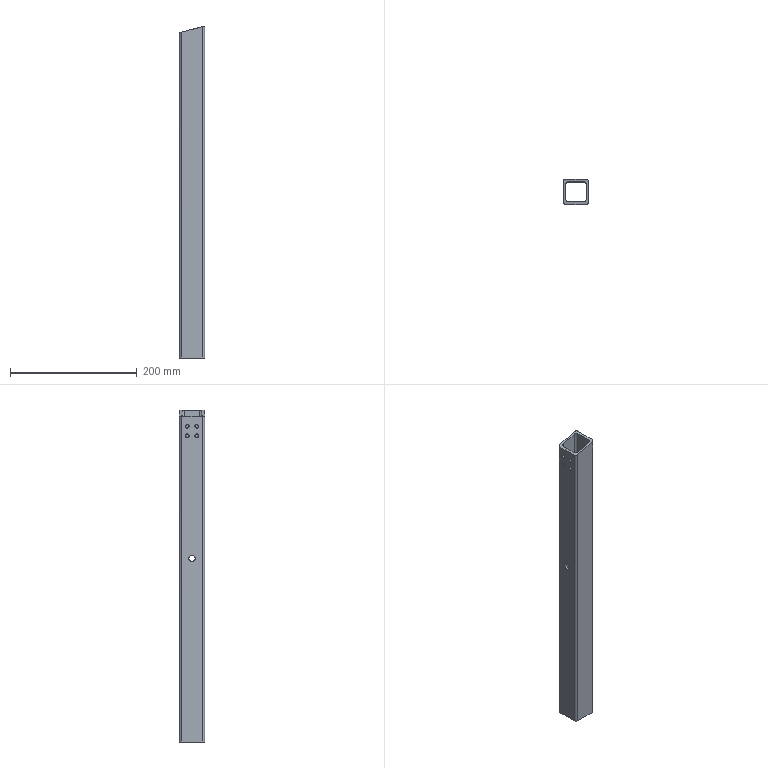Component | NX | SLANT_VERT_ROD_1_2 | 1 solid | 32 faces | volume 298124 mm3 | cylinder 14 | plane 10 | cone 8 | commonest cylinder face diameters 8 x8 5 x4 10 x2